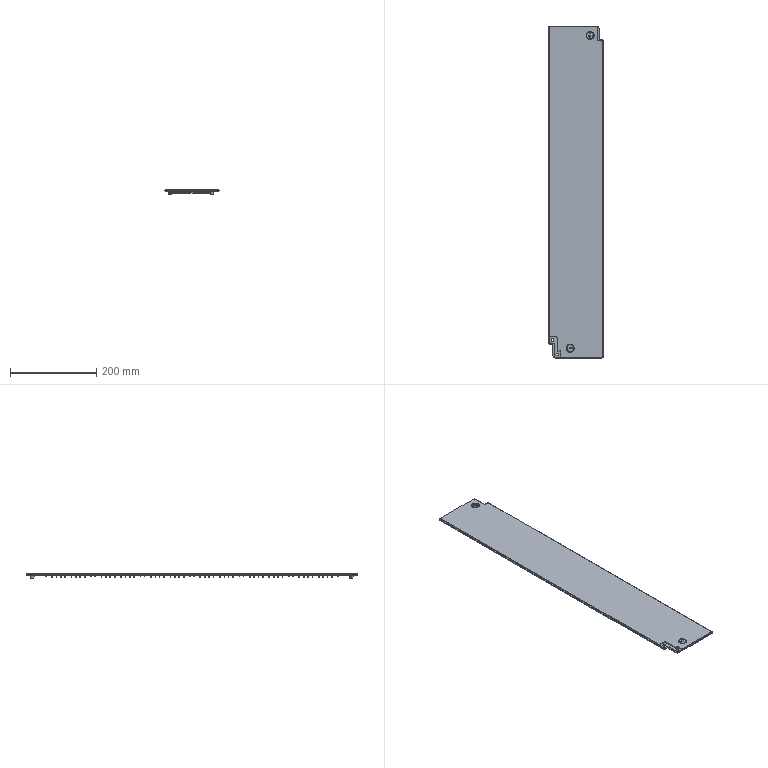Component | SolidWorks | Cover-glzt-xin.0310-1 | 2 solids | 560 faces | volume 404229 mm3 | plane 501 | cylinder 49 | cone 7 | spline 3 | commonest cylinder face diameters 3.2 x13 7 x12 6.3 x6 15.9 x6 19.1 x4 9.6 x4 11 x2 12.9 x2